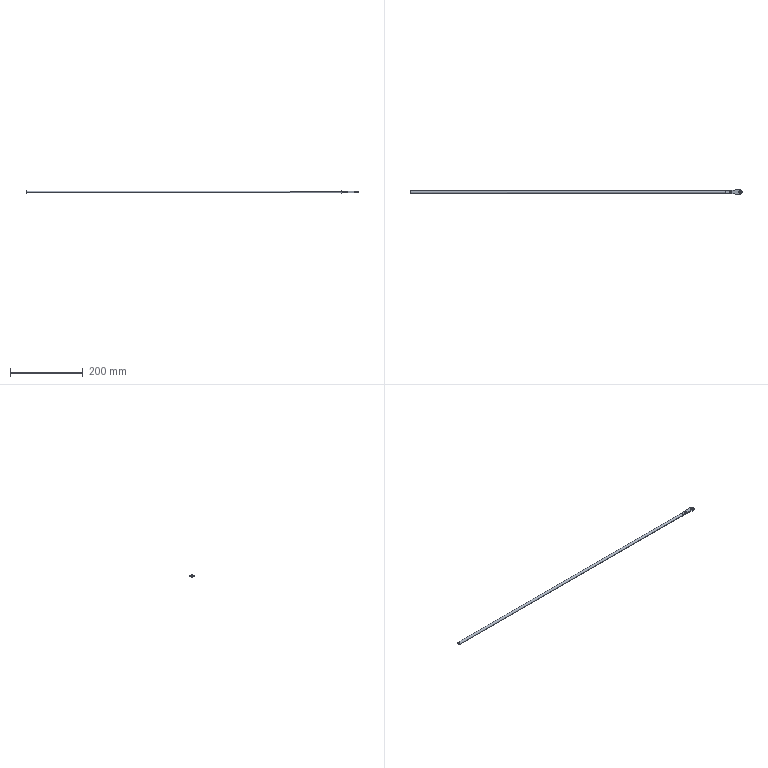Component | SolidWorks | RightRearDoorFrameAssembly-1_RearDoorUpperLockRod-1 | 1 solid | 20 faces | box 912.5 x 13 x 8 mm | volume 44809 mm3 | plane 11 | cylinder 7 | cone 2 | commonest cylinder face diameters 6.5 x4 8 x2 13 x1
build123d program:
from build123d import *

# Parameters (mm, degrees)
SKETCH1_R           = 4
BOSS_EXTRUDE1_DEPTH = 912.5
CUT_EXTRUDE1_DEPTH  = 5
SKETCH3_W           = 42
SKETCH3_H           = 2.024
CUT_EXTRUDE2_DEPTH  = 10
BOSS_EXTRUDE2_DEPTH = 3
CUT_EXTRUDE3_DEPTH  = 3
SKETCH6_R           = 3.25
CUT_EXTRUDE4_DEPTH  = 3
CHAMFER1_SIZE       = 1.5


with BuildPart() as part:
    # Sketch1 → Boss-Extrude1 (new body)
    with BuildSketch(Plane(origin=(0, 0, 0), x_dir=(0, 0, -1), z_dir=(1, 0, 0))):
        Circle(SKETCH1_R)
    extrude(amount=-BOSS_EXTRUDE1_DEPTH)

    # Sketch2 → Cut-Extrude1 (cut, symmetric)
    with BuildSketch(Plane.XY):
        Polygon((-42, 1.5), (-45.678, 4), (-42, 4), (0, 4), (0, 1.5), align=None)
        Polygon((-45.678, -4), (-42, -4), (0, -4), (0, -1.5), (-42, -1.5), align=None)
    extrude(amount=CUT_EXTRUDE1_DEPTH, both=True, mode=Mode.SUBTRACT)

    # Sketch3 → Cut-Extrude2 (cut)
    with BuildSketch(Plane(origin=(0, 1.5, 0), x_dir=(1, 0, 0), z_dir=(0, 1, 0))):
        with Locations((-21, 2.988)):
            Rectangle(SKETCH3_W, SKETCH3_H)
        with Locations((-21, -2.988)):
            Rectangle(SKETCH3_W, SKETCH3_H)
    extrude(amount=-CUT_EXTRUDE2_DEPTH, mode=Mode.SUBTRACT)

    # Sketch4 → Boss-Extrude2 (add)
    with BuildSketch(Plane(origin=(0, 1.5, 0), x_dir=(1, 0, 0), z_dir=(0, 1, 0))):
        with BuildLine():
            Line((-42, -4), (-42, 4))
            Line((-42, 4), (-7.386, 6.439))
            ThreePointArc((-7.386, 6.439), (0, 0), (-7.386, -6.439))
            Line((-7.386, -6.439), (-42, -4))
        make_face()
    extrude(amount=-BOSS_EXTRUDE2_DEPTH)

    # Sketch5 → Cut-Extrude3 (cut)
    with BuildSketch(Plane(origin=(0, 1.5, 0), x_dir=(1, 0, 0), z_dir=(0, 1, 0))):
        with BuildLine():
            Line((-0.8017, 3.127), (2.344, 3.127))
            Line((2.344, 3.127), (2.344, -3.404))
            Line((2.344, -3.404), (-0.9628, -3.404))
            ThreePointArc((-0.9628, -3.404), (-0.001977, -0.1603), (-0.8017, 3.127))
        make_face()
    extrude(amount=-CUT_EXTRUDE3_DEPTH, mode=Mode.SUBTRACT)

    # Sketch6 → Cut-Extrude4 (cut)
    with BuildSketch(Plane(origin=(0, 1.5, 0), x_dir=(1, 0, 0), z_dir=(0, 1, 0))):
        with Locations(Location((-6, 0, 0), (0, 0, 180))):
            Circle(SKETCH6_R)
        with Locations(Location((-31, 0, 0), (0, 0, 180))):
            Circle(SKETCH6_R)
    extrude(amount=-CUT_EXTRUDE4_DEPTH, mode=Mode.SUBTRACT)

    # Chamfer1
    chamfer1_edges = [part.edges().sort_by_distance(p)[0] for p in [
        (-912.5, 0, 4),
    ]]
    chamfer(chamfer1_edges, length=CHAMFER1_SIZE)


solid = part.part

# Placed as in the assembly
solid = solid.moved(Location((-209.186, 303.707, -28.746), (90, 0, 0)))
STEP:
#1=COLOUR_RGB('',0.7922,0.8196,0.9333);
#2=FILL_AREA_STYLE_COLOUR('',#1);
#3=FILL_AREA_STYLE('',(#2));
#4=SURFACE_STYLE_FILL_AREA(#3);
#5=SURFACE_SIDE_STYLE('',(#4));
#6=SURFACE_STYLE_USAGE(.BOTH.,#5);
#7=PRESENTATION_STYLE_ASSIGNMENT((#6));
#8=CARTESIAN_POINT('',(-44.161,12.055,-1.132));
#9=VERTEX_POINT('',#8);
#10=CARTESIAN_POINT('',(-44.161,11.859,-1.132));
#11=VERTEX_POINT('',#10);
#12=CARTESIAN_POINT('',(-44.161,11.957,-1.132));
#13=DIRECTION('',(-1.,-0.,-0.));
#14=DIRECTION('',(0.,-1.,0.));
#15=AXIS2_PLACEMENT_3D('',#12,#13,#14);
#16=CIRCLE('',#15,0.09843);
#17=EDGE_CURVE('',#9,#11,#16,.T.);
#18=ORIENTED_EDGE('',*,*,#17,.F.);
#19=CARTESIAN_POINT('',(-44.102,12.114,-1.132));
#20=VERTEX_POINT('',#19);
#21=CARTESIAN_POINT('',(-44.102,12.114,-1.132));
#22=DIRECTION('',(0.7071,0.7071,0.));
#23=VECTOR('',#22,39.37);
#24=LINE('',#21,#23);
#25=EDGE_CURVE('',#9,#20,#24,.T.);
#26=ORIENTED_EDGE('',*,*,#25,.T.);
#27=CARTESIAN_POINT('',(-44.102,11.799,-1.132));
#28=VERTEX_POINT('',#27);
#29=CARTESIAN_POINT('',(-44.102,11.957,-1.132));
#30=DIRECTION('',(1.,0.,0.));
#31=DIRECTION('',(0.,-1.,0.));
#32=AXIS2_PLACEMENT_3D('',#29,#30,#31);
#33=CIRCLE('',#32,0.1575);
#34=EDGE_CURVE('',#28,#20,#33,.T.);
#35=ORIENTED_EDGE('',*,*,#34,.F.);
#36=CARTESIAN_POINT('',(-44.102,11.799,-1.132));
#37=DIRECTION('',(0.7071,-0.7071,0.));
#38=VECTOR('',#37,39.37);
#39=LINE('',#36,#38);
#40=EDGE_CURVE('',#11,#28,#39,.T.);
#41=ORIENTED_EDGE('',*,*,#40,.F.);
#42=EDGE_LOOP('',(#18,#26,#35,#41));
#43=FACE_OUTER_BOUND('',#42,.T.);
#44=CARTESIAN_POINT('',(-44.102,11.957,-1.132));
#45=DIRECTION('',(1.,0.,0.));
#46=DIRECTION('',(0.,-1.,0.));
#47=AXIS2_PLACEMENT_3D('',#44,#45,#46);
#48=CONICAL_SURFACE('',#47,0.1575,0.7854);
#49=ADVANCED_FACE('',(#43),#48,.T.);
#50=CARTESIAN_POINT('',(-9.328,11.957,-1.073));
#51=VERTEX_POINT('',#50);
#52=CARTESIAN_POINT('',(-9.584,11.957,-1.073));
#53=VERTEX_POINT('',#52);
#54=CARTESIAN_POINT('',(-9.456,11.957,-1.073));
#55=DIRECTION('',(0.,0.,-1.));
#56=DIRECTION('',(-1.,0.,0.));
#57=AXIS2_PLACEMENT_3D('',#54,#55,#56);
#58=CIRCLE('',#57,0.128);
#59=EDGE_CURVE('',#51,#53,#58,.T.);
#60=ORIENTED_EDGE('',*,*,#59,.F.);
#61=CARTESIAN_POINT('',(-9.328,11.957,-1.191));
#62=VERTEX_POINT('',#61);
#63=CARTESIAN_POINT('',(-9.328,11.957,-1.073));
#64=DIRECTION('',(0.,0.,-1.));
#65=VECTOR('',#64,39.37);
#66=LINE('',#63,#65);
#67=EDGE_CURVE('',#51,#62,#66,.T.);
#68=ORIENTED_EDGE('',*,*,#67,.T.);
#69=CARTESIAN_POINT('',(-9.584,11.957,-1.191));
#70=VERTEX_POINT('',#69);
#71=CARTESIAN_POINT('',(-9.456,11.957,-1.191));
#72=DIRECTION('',(0.,0.,-1.));
#73=DIRECTION('',(-1.,0.,0.));
#74=AXIS2_PLACEMENT_3D('',#71,#72,#73);
#75=CIRCLE('',#74,0.128);
#76=EDGE_CURVE('',#62,#70,#75,.T.);
#77=ORIENTED_EDGE('',*,*,#76,.T.);
#78=CARTESIAN_POINT('',(-9.584,11.957,-1.073));
#79=DIRECTION('',(0.,0.,-1.));
#80=VECTOR('',#79,39.37);
#81=LINE('',#78,#80);
#82=EDGE_CURVE('',#53,#70,#81,.T.);
#83=ORIENTED_EDGE('',*,*,#82,.F.);
#84=EDGE_LOOP('',(#60,#68,#77,#83));
#85=FACE_OUTER_BOUND('',#84,.T.);
#86=CARTESIAN_POINT('',(-9.456,11.957,-1.073));
#87=DIRECTION('',(0.,0.,-1.));
#88=DIRECTION('',(-1.,0.,0.));
#89=AXIS2_PLACEMENT_3D('',#86,#87,#88);
#90=CYLINDRICAL_SURFACE('',#89,0.128);
#91=ADVANCED_FACE('',(#85),#90,.F.);
#92=CARTESIAN_POINT('',(-8.344,11.957,-1.073));
#93=VERTEX_POINT('',#92);
#94=CARTESIAN_POINT('',(-8.6,11.957,-1.073));
#95=VERTEX_POINT('',#94);
#96=CARTESIAN_POINT('',(-8.472,11.957,-1.073));
#97=DIRECTION('',(0.,0.,-1.));
#98=DIRECTION('',(-1.,0.,0.));
#99=AXIS2_PLACEMENT_3D('',#96,#97,#98);
#100=CIRCLE('',#99,0.128);
#101=EDGE_CURVE('',#93,#95,#100,.T.);
#102=ORIENTED_EDGE('',*,*,#101,.F.);
#103=CARTESIAN_POINT('',(-8.344,11.957,-1.191));
#104=VERTEX_POINT('',#103);
#105=CARTESIAN_POINT('',(-8.344,11.957,-1.073));
#106=DIRECTION('',(0.,0.,-1.));
#107=VECTOR('',#106,39.37);
#108=LINE('',#105,#107);
#109=EDGE_CURVE('',#93,#104,#108,.T.);
#110=ORIENTED_EDGE('',*,*,#109,.T.);
#111=CARTESIAN_POINT('',(-8.6,11.957,-1.191));
#112=VERTEX_POINT('',#111);
#113=CARTESIAN_POINT('',(-8.472,11.957,-1.191));
#114=DIRECTION('',(0.,0.,-1.));
#115=DIRECTION('',(-1.,0.,0.));
#116=AXIS2_PLACEMENT_3D('',#113,#114,#115);
#117=CIRCLE('',#116,0.128);
#118=EDGE_CURVE('',#104,#112,#117,.T.);
#119=ORIENTED_EDGE('',*,*,#118,.T.);
#120=CARTESIAN_POINT('',(-8.6,11.957,-1.073));
#121=DIRECTION('',(0.,0.,-1.));
#122=VECTOR('',#121,39.37);
#123=LINE('',#120,#122);
#124=EDGE_CURVE('',#95,#112,#123,.T.);
#125=ORIENTED_EDGE('',*,*,#124,.F.);
#126=EDGE_LOOP('',(#102,#110,#119,#125));
#127=FACE_OUTER_BOUND('',#126,.T.);
#128=CARTESIAN_POINT('',(-8.472,11.957,-1.073));
#129=DIRECTION('',(0.,0.,-1.));
#130=DIRECTION('',(-1.,0.,0.));
#131=AXIS2_PLACEMENT_3D('',#128,#129,#130);
#132=CYLINDRICAL_SURFACE('',#131,0.128);
#133=ADVANCED_FACE('',(#127),#132,.F.);
#134=ORIENTED_EDGE('',*,*,#34,.T.);
#135=CARTESIAN_POINT('',(-9.889,12.114,-1.132));
#136=VERTEX_POINT('',#135);
#137=CARTESIAN_POINT('',(-44.161,12.114,-1.132));
#138=DIRECTION('',(1.,0.,0.));
#139=VECTOR('',#138,39.37);
#140=LINE('',#137,#139);
#141=EDGE_CURVE('',#20,#136,#140,.T.);
#142=ORIENTED_EDGE('',*,*,#141,.T.);
#143=CARTESIAN_POINT('',(-9.889,12.103,-1.191));
#144=VERTEX_POINT('',#143);
#145=CARTESIAN_POINT('',(-9.889,11.957,-1.132));
#146=DIRECTION('',(1.,0.,0.));
#147=DIRECTION('',(0.,-0.,1.));
#148=AXIS2_PLACEMENT_3D('',#145,#146,#147);
#149=CIRCLE('',#148,0.1575);
#150=EDGE_CURVE('',#144,#136,#149,.T.);
#151=ORIENTED_EDGE('',*,*,#150,.F.);
#152=CARTESIAN_POINT('',(-9.889,11.811,-1.191));
#153=VERTEX_POINT('',#152);
#154=CARTESIAN_POINT('',(-9.889,11.811,-1.191));
#155=CARTESIAN_POINT('',(-10.117,11.874,-1.345));
#156=CARTESIAN_POINT('',(-10.117,12.04,-1.345));
#157=CARTESIAN_POINT('',(-9.889,12.103,-1.191));
#158=(BOUNDED_CURVE()B_SPLINE_CURVE(3,(#154,#155,#156,#157),.UNSPECIFIED.,.F.,.T.)B_SPLINE_CURVE_WITH_KNOTS((4,4),(1.955,4.328),.UNSPECIFIED.)CURVE()GEOMETRIC_REPRESENTATION_ITEM()RATIONAL_B_SPLINE_CURVE((1.,0.5833,0.5833,1.))REPRESENTATION_ITEM(''));
#159=EDGE_CURVE('',#153,#144,#158,.T.);
#160=ORIENTED_EDGE('',*,*,#159,.F.);
#161=CARTESIAN_POINT('',(-9.889,11.799,-1.132));
#162=VERTEX_POINT('',#161);
#163=CARTESIAN_POINT('',(-9.889,11.957,-1.132));
#164=DIRECTION('',(1.,0.,0.));
#165=DIRECTION('',(0.,-0.,1.));
#166=AXIS2_PLACEMENT_3D('',#163,#164,#165);
#167=CIRCLE('',#166,0.1575);
#168=EDGE_CURVE('',#162,#153,#167,.T.);
#169=ORIENTED_EDGE('',*,*,#168,.F.);
#170=CARTESIAN_POINT('',(-44.161,11.799,-1.132));
#171=DIRECTION('',(1.,0.,0.));
#172=VECTOR('',#171,39.37);
#173=LINE('',#170,#172);
#174=EDGE_CURVE('',#28,#162,#173,.T.);
#175=ORIENTED_EDGE('',*,*,#174,.F.);
#176=EDGE_LOOP('',(#134,#142,#151,#160,#169,#175));
#177=FACE_OUTER_BOUND('',#176,.T.);
#178=CARTESIAN_POINT('',(-44.161,11.957,-1.132));
#179=DIRECTION('',(1.,0.,0.));
#180=DIRECTION('',(0.,-1.,0.));
#181=AXIS2_PLACEMENT_3D('',#178,#179,#180);
#182=CYLINDRICAL_SURFACE('',#181,0.1575);
#183=ADVANCED_FACE('',(#177),#182,.T.);
#184=ORIENTED_EDGE('',*,*,#141,.F.);
#185=CARTESIAN_POINT('',(-44.102,11.957,-1.132));
#186=DIRECTION('',(1.,0.,0.));
#187=DIRECTION('',(0.,-1.,0.));
#188=AXIS2_PLACEMENT_3D('',#185,#186,#187);
#189=CIRCLE('',#188,0.1575);
#190=EDGE_CURVE('',#20,#28,#189,.T.);
#191=ORIENTED_EDGE('',*,*,#190,.T.);
#192=ORIENTED_EDGE('',*,*,#174,.T.);
#193=CARTESIAN_POINT('',(-9.889,11.811,-1.073));
#194=VERTEX_POINT('',#193);
#195=CARTESIAN_POINT('',(-9.889,11.957,-1.132));
#196=DIRECTION('',(1.,0.,0.));
#197=DIRECTION('',(0.,-0.,1.));
#198=AXIS2_PLACEMENT_3D('',#195,#196,#197);
#199=CIRCLE('',#198,0.1575);
#200=EDGE_CURVE('',#194,#162,#199,.T.);
#201=ORIENTED_EDGE('',*,*,#200,.F.);
#202=CARTESIAN_POINT('',(-9.889,12.103,-1.073));
#203=VERTEX_POINT('',#202);
#204=CARTESIAN_POINT('',(-9.889,12.103,-1.073));
#205=CARTESIAN_POINT('',(-10.117,12.04,-0.918));
#206=CARTESIAN_POINT('',(-10.117,11.874,-0.918));
#207=CARTESIAN_POINT('',(-9.889,11.811,-1.073));
#208=(BOUNDED_CURVE()B_SPLINE_CURVE(3,(#204,#205,#206,#207),.UNSPECIFIED.,.F.,.F.)B_SPLINE_CURVE_WITH_KNOTS((4,4),(1.955,4.328),.UNSPECIFIED.)CURVE()GEOMETRIC_REPRESENTATION_ITEM()RATIONAL_B_SPLINE_CURVE((1.,0.5833,0.5833,1.))REPRESENTATION_ITEM(''));
#209=EDGE_CURVE('',#203,#194,#208,.T.);
#210=ORIENTED_EDGE('',*,*,#209,.F.);
#211=CARTESIAN_POINT('',(-9.889,11.957,-1.132));
#212=DIRECTION('',(1.,0.,0.));
#213=DIRECTION('',(0.,0.,1.));
#214=AXIS2_PLACEMENT_3D('',#211,#212,#213);
#215=CIRCLE('',#214,0.1575);
#216=EDGE_CURVE('',#136,#203,#215,.T.);
#217=ORIENTED_EDGE('',*,*,#216,.F.);
#218=EDGE_LOOP('',(#184,#191,#192,#201,#210,#217));
#219=FACE_OUTER_BOUND('',#218,.T.);
#220=CARTESIAN_POINT('',(-44.161,11.957,-1.132));
#221=DIRECTION('',(1.,0.,0.));
#222=DIRECTION('',(0.,-1.,0.));
#223=AXIS2_PLACEMENT_3D('',#220,#221,#222);
#224=CYLINDRICAL_SURFACE('',#223,0.1575);
#225=ADVANCED_FACE('',(#219),#224,.T.);
#226=CARTESIAN_POINT('',(-44.161,11.957,-1.132));
#227=DIRECTION('',(-1.,-0.,-0.));
#228=DIRECTION('',(0.,-1.,0.));
#229=AXIS2_PLACEMENT_3D('',#226,#227,#228);
#230=CIRCLE('',#229,0.09843);
#231=EDGE_CURVE('',#11,#9,#230,.T.);
#232=ORIENTED_EDGE('',*,*,#231,.T.);
#233=ORIENTED_EDGE('',*,*,#17,.T.);
#234=EDGE_LOOP('',(#232,#233));
#235=FACE_OUTER_BOUND('',#234,.T.);
#236=CARTESIAN_POINT('',(-44.161,11.957,-1.132));
#237=DIRECTION('',(1.,0.,0.));
#238=DIRECTION('',(0.,-1.,-0.));
#239=AXIS2_PLACEMENT_3D('',#236,#237,#238);
#240=PLANE('',#239);
#241=ADVANCED_FACE('',(#235),#240,.F.);
#242=CARTESIAN_POINT('',(-9.456,11.957,-1.191));
#243=DIRECTION('',(0.,0.,-1.));
#244=DIRECTION('',(-1.,0.,0.));
#245=AXIS2_PLACEMENT_3D('',#242,#243,#244);
#246=CIRCLE('',#245,0.128);
#247=EDGE_CURVE('',#70,#62,#246,.T.);
#248=ORIENTED_EDGE('',*,*,#247,.F.);
#249=ORIENTED_EDGE('',*,*,#76,.F.);
#250=EDGE_LOOP('',(#248,#249));
#251=FACE_BOUND('',#250,.T.);
#252=CARTESIAN_POINT('',(-8.472,11.957,-1.191));
#253=DIRECTION('',(0.,0.,-1.));
#254=DIRECTION('',(-1.,0.,0.));
#255=AXIS2_PLACEMENT_3D('',#252,#253,#254);
#256=CIRCLE('',#255,0.128);
#257=EDGE_CURVE('',#112,#104,#256,.T.);
#258=ORIENTED_EDGE('',*,*,#257,.F.);
#259=ORIENTED_EDGE('',*,*,#118,.F.);
#260=EDGE_LOOP('',(#258,#259));
#261=FACE_BOUND('',#260,.T.);
#262=CARTESIAN_POINT('',(-9.889,12.114,-1.191));
#263=VERTEX_POINT('',#262);
#264=CARTESIAN_POINT('',(-8.526,12.21,-1.191));
#265=VERTEX_POINT('',#264);
#266=CARTESIAN_POINT('',(-9.889,12.114,-1.191));
#267=DIRECTION('',(0.9975,0.0703,0.));
#268=VECTOR('',#267,39.37);
#269=LINE('',#266,#268);
#270=EDGE_CURVE('',#263,#265,#269,.T.);
#271=ORIENTED_EDGE('',*,*,#270,.T.);
#272=CARTESIAN_POINT('',(-8.526,11.703,-1.191));
#273=VERTEX_POINT('',#272);
#274=CARTESIAN_POINT('',(-8.492,11.957,-1.191));
#275=DIRECTION('',(0.,0.,-1.));
#276=DIRECTION('',(-1.,0.,0.));
#277=AXIS2_PLACEMENT_3D('',#274,#275,#276);
#278=CIRCLE('',#277,0.2559);
#279=EDGE_CURVE('',#265,#273,#278,.T.);
#280=ORIENTED_EDGE('',*,*,#279,.T.);
#281=CARTESIAN_POINT('',(-9.889,11.799,-1.191));
#282=VERTEX_POINT('',#281);
#283=CARTESIAN_POINT('',(-9.889,11.799,-1.191));
#284=DIRECTION('',(-0.9975,0.0703,-0.));
#285=VECTOR('',#284,39.37);
#286=LINE('',#283,#285);
#287=EDGE_CURVE('',#273,#282,#286,.T.);
#288=ORIENTED_EDGE('',*,*,#287,.T.);
#289=CARTESIAN_POINT('',(-9.889,12.114,-1.191));
#290=DIRECTION('',(-0.,1.,0.));
#291=VECTOR('',#290,39.37);
#292=LINE('',#289,#291);
#293=EDGE_CURVE('',#282,#153,#292,.T.);
#294=ORIENTED_EDGE('',*,*,#293,.T.);
#295=CARTESIAN_POINT('',(-9.889,11.76,-1.191));
#296=DIRECTION('',(-0.,1.,0.));
#297=VECTOR('',#296,39.37);
#298=LINE('',#295,#297);
#299=EDGE_CURVE('',#153,#144,#298,.T.);
#300=ORIENTED_EDGE('',*,*,#299,.T.);
#301=CARTESIAN_POINT('',(-9.889,12.114,-1.191));
#302=DIRECTION('',(-0.,1.,0.));
#303=VECTOR('',#302,39.37);
#304=LINE('',#301,#303);
#305=EDGE_CURVE('',#144,#263,#304,.T.);
#306=ORIENTED_EDGE('',*,*,#305,.T.);
#307=EDGE_LOOP('',(#271,#280,#288,#294,#300,#306));
#308=FACE_OUTER_BOUND('',#307,.T.);
#309=CARTESIAN_POINT('',(-8.236,11.76,-1.191));
#310=DIRECTION('',(-0.,-0.,1.));
#311=DIRECTION('',(1.,0.,0.));
#312=AXIS2_PLACEMENT_3D('',#309,#310,#311);
#313=PLANE('',#312);
#314=ADVANCED_FACE('',(#251,#261,#308),#313,.F.);
#315=ORIENTED_EDGE('',*,*,#299,.F.);
#316=ORIENTED_EDGE('',*,*,#159,.T.);
#317=EDGE_LOOP('',(#315,#316));
#318=FACE_OUTER_BOUND('',#317,.T.);
#319=CARTESIAN_POINT('',(-9.889,11.76,-1.191));
#320=DIRECTION('',(-0.5621,-0.,0.8271));
#321=DIRECTION('',(0.8271,0.,0.5621));
#322=AXIS2_PLACEMENT_3D('',#319,#320,#321);
#323=PLANE('',#322);
#324=ADVANCED_FACE('',(#318),#323,.F.);
#325=CARTESIAN_POINT('',(-9.889,11.76,-1.073));
#326=DIRECTION('',(-0.,1.,0.));
#327=VECTOR('',#326,39.37);
#328=LINE('',#325,#327);
#329=EDGE_CURVE('',#194,#203,#328,.T.);
#330=ORIENTED_EDGE('',*,*,#329,.T.);
#331=ORIENTED_EDGE('',*,*,#209,.T.);
#332=EDGE_LOOP('',(#330,#331));
#333=FACE_OUTER_BOUND('',#332,.T.);
#334=CARTESIAN_POINT('',(-9.889,11.76,-1.073));
#335=DIRECTION('',(-0.5621,-0.,-0.8271));
#336=DIRECTION('',(-0.8271,-0.,0.5621));
#337=AXIS2_PLACEMENT_3D('',#334,#335,#336);
#338=PLANE('',#337);
#339=ADVANCED_FACE('',(#333),#338,.F.);
#340=CARTESIAN_POINT('',(-9.456,11.957,-1.073));
#341=DIRECTION('',(0.,0.,-1.));
#342=DIRECTION('',(-1.,0.,0.));
#343=AXIS2_PLACEMENT_3D('',#340,#341,#342);
#344=CIRCLE('',#343,0.128);
#345=EDGE_CURVE('',#53,#51,#344,.T.);
#346=ORIENTED_EDGE('',*,*,#345,.T.);
#347=ORIENTED_EDGE('',*,*,#59,.T.);
#348=EDGE_LOOP('',(#346,#347));
#349=FACE_BOUND('',#348,.T.);
#350=CARTESIAN_POINT('',(-8.472,11.957,-1.073));
#351=DIRECTION('',(0.,0.,-1.));
#352=DIRECTION('',(-1.,0.,0.));
#353=AXIS2_PLACEMENT_3D('',#350,#351,#352);
#354=CIRCLE('',#353,0.128);
#355=EDGE_CURVE('',#95,#93,#354,.T.);
#356=ORIENTED_EDGE('',*,*,#355,.T.);
#357=ORIENTED_EDGE('',*,*,#101,.T.);
#358=EDGE_LOOP('',(#356,#357));
#359=FACE_BOUND('',#358,.T.);
#360=CARTESIAN_POINT('',(-8.526,12.21,-1.073));
#361=VERTEX_POINT('',#360);
#362=CARTESIAN_POINT('',(-8.526,11.703,-1.073));
#363=VERTEX_POINT('',#362);
#364=CARTESIAN_POINT('',(-8.492,11.957,-1.073));
#365=DIRECTION('',(0.,0.,-1.));
#366=DIRECTION('',(-1.,0.,0.));
#367=AXIS2_PLACEMENT_3D('',#364,#365,#366);
#368=CIRCLE('',#367,0.2559);
#369=EDGE_CURVE('',#361,#363,#368,.T.);
#370=ORIENTED_EDGE('',*,*,#369,.F.);
#371=CARTESIAN_POINT('',(-9.889,12.114,-1.073));
#372=VERTEX_POINT('',#371);
#373=CARTESIAN_POINT('',(-9.889,12.114,-1.073));
#374=DIRECTION('',(0.9975,0.0703,0.));
#375=VECTOR('',#374,39.37);
#376=LINE('',#373,#375);
#377=EDGE_CURVE('',#372,#361,#376,.T.);
#378=ORIENTED_EDGE('',*,*,#377,.F.);
#379=CARTESIAN_POINT('',(-9.889,12.114,-1.073));
#380=DIRECTION('',(-0.,1.,0.));
#381=VECTOR('',#380,39.37);
#382=LINE('',#379,#381);
#383=EDGE_CURVE('',#203,#372,#382,.T.);
#384=ORIENTED_EDGE('',*,*,#383,.F.);
#385=ORIENTED_EDGE('',*,*,#329,.F.);
#386=CARTESIAN_POINT('',(-9.889,11.799,-1.073));
#387=VERTEX_POINT('',#386);
#388=CARTESIAN_POINT('',(-9.889,12.114,-1.073));
#389=DIRECTION('',(-0.,1.,0.));
#390=VECTOR('',#389,39.37);
#391=LINE('',#388,#390);
#392=EDGE_CURVE('',#387,#194,#391,.T.);
#393=ORIENTED_EDGE('',*,*,#392,.F.);
#394=CARTESIAN_POINT('',(-9.889,11.799,-1.073));
#395=DIRECTION('',(-0.9975,0.0703,-0.));
#396=VECTOR('',#395,39.37);
#397=LINE('',#394,#396);
#398=EDGE_CURVE('',#363,#387,#397,.T.);
#399=ORIENTED_EDGE('',*,*,#398,.F.);
#400=EDGE_LOOP('',(#370,#378,#384,#385,#393,#399));
#401=FACE_OUTER_BOUND('',#400,.T.);
#402=CARTESIAN_POINT('',(-8.236,11.76,-1.073));
#403=DIRECTION('',(0.,0.,-1.));
#404=DIRECTION('',(-1.,-0.,-0.));
#405=AXIS2_PLACEMENT_3D('',#402,#403,#404);
#406=PLANE('',#405);
#407=ADVANCED_FACE('',(#349,#359,#401),#406,.F.);
#408=ORIENTED_EDGE('',*,*,#270,.F.);
#409=CARTESIAN_POINT('',(-9.889,12.114,-1.073));
#410=DIRECTION('',(0.,0.,-1.));
#411=VECTOR('',#410,39.37);
#412=LINE('',#409,#411);
#413=EDGE_CURVE('',#136,#263,#412,.T.);
#414=ORIENTED_EDGE('',*,*,#413,.F.);
#415=CARTESIAN_POINT('',(-9.889,12.114,-1.073));
#416=DIRECTION('',(0.,0.,-1.));
#417=VECTOR('',#416,39.37);
#418=LINE('',#415,#417);
#419=EDGE_CURVE('',#372,#136,#418,.T.);
#420=ORIENTED_EDGE('',*,*,#419,.F.);
#421=ORIENTED_EDGE('',*,*,#377,.T.);
#422=CARTESIAN_POINT('',(-8.526,12.21,-1.073));
#423=DIRECTION('',(0.,0.,-1.));
#424=VECTOR('',#423,39.37);
#425=LINE('',#422,#424);
#426=EDGE_CURVE('',#361,#265,#425,.T.);
#427=ORIENTED_EDGE('',*,*,#426,.T.);
#428=EDGE_LOOP('',(#408,#414,#420,#421,#427));
#429=FACE_OUTER_BOUND('',#428,.T.);
#430=CARTESIAN_POINT('',(-9.889,12.114,-1.073));
#431=DIRECTION('',(-0.0703,0.9975,0.));
#432=DIRECTION('',(0.9975,0.0703,0.));
#433=AXIS2_PLACEMENT_3D('',#430,#431,#432);
#434=PLANE('',#433);
#435=ADVANCED_FACE('',(#429),#434,.T.);
#436=ORIENTED_EDGE('',*,*,#419,.T.);
#437=ORIENTED_EDGE('',*,*,#216,.T.);
#438=ORIENTED_EDGE('',*,*,#383,.T.);
#439=EDGE_LOOP('',(#436,#437,#438));
#440=FACE_OUTER_BOUND('',#439,.T.);
#441=CARTESIAN_POINT('',(-9.889,12.114,-1.073));
#442=DIRECTION('',(-1.,-0.,-0.));
#443=DIRECTION('',(-0.,-0.,1.));
#444=AXIS2_PLACEMENT_3D('',#441,#442,#443);
#445=PLANE('',#444);
#446=ADVANCED_FACE('',(#440),#445,.T.);
#447=ORIENTED_EDGE('',*,*,#305,.F.);
#448=ORIENTED_EDGE('',*,*,#150,.T.);
#449=ORIENTED_EDGE('',*,*,#413,.T.);
#450=EDGE_LOOP('',(#447,#448,#449));
#451=FACE_OUTER_BOUND('',#450,.T.);
#452=CARTESIAN_POINT('',(-9.889,12.114,-1.073));
#453=DIRECTION('',(-1.,-0.,-0.));
#454=DIRECTION('',(-0.,-0.,1.));
#455=AXIS2_PLACEMENT_3D('',#452,#453,#454);
#456=PLANE('',#455);
#457=ADVANCED_FACE('',(#451),#456,.T.);
#458=ORIENTED_EDGE('',*,*,#392,.T.);
#459=ORIENTED_EDGE('',*,*,#200,.T.);
#460=CARTESIAN_POINT('',(-9.889,11.799,-1.073));
#461=DIRECTION('',(0.,0.,-1.));
#462=VECTOR('',#461,39.37);
#463=LINE('',#460,#462);
#464=EDGE_CURVE('',#387,#162,#463,.T.);
#465=ORIENTED_EDGE('',*,*,#464,.F.);
#466=EDGE_LOOP('',(#458,#459,#465));
#467=FACE_OUTER_BOUND('',#466,.T.);
#468=CARTESIAN_POINT('',(-9.889,12.114,-1.073));
#469=DIRECTION('',(-1.,-0.,-0.));
#470=DIRECTION('',(-0.,-0.,1.));
#471=AXIS2_PLACEMENT_3D('',#468,#469,#470);
#472=PLANE('',#471);
#473=ADVANCED_FACE('',(#467),#472,.T.);
#474=CARTESIAN_POINT('',(-9.889,11.799,-1.073));
#475=DIRECTION('',(0.,0.,-1.));
#476=VECTOR('',#475,39.37);
#477=LINE('',#474,#476);
#478=EDGE_CURVE('',#162,#282,#477,.T.);
#479=ORIENTED_EDGE('',*,*,#478,.F.);
#480=ORIENTED_EDGE('',*,*,#168,.T.);
#481=ORIENTED_EDGE('',*,*,#293,.F.);
#482=EDGE_LOOP('',(#479,#480,#481));
#483=FACE_OUTER_BOUND('',#482,.T.);
#484=CARTESIAN_POINT('',(-9.889,12.114,-1.073));
#485=DIRECTION('',(-1.,-0.,-0.));
#486=DIRECTION('',(-0.,-0.,1.));
#487=AXIS2_PLACEMENT_3D('',#484,#485,#486);
#488=PLANE('',#487);
#489=ADVANCED_FACE('',(#483),#488,.T.);
#490=CARTESIAN_POINT('',(-8.526,11.703,-1.073));
#491=DIRECTION('',(0.,0.,-1.));
#492=VECTOR('',#491,39.37);
#493=LINE('',#490,#492);
#494=EDGE_CURVE('',#363,#273,#493,.T.);
#495=ORIENTED_EDGE('',*,*,#494,.T.);
#496=ORIENTED_EDGE('',*,*,#279,.F.);
#497=ORIENTED_EDGE('',*,*,#426,.F.);
#498=ORIENTED_EDGE('',*,*,#369,.T.);
#499=EDGE_LOOP('',(#495,#496,#497,#498));
#500=FACE_OUTER_BOUND('',#499,.T.);
#501=CARTESIAN_POINT('',(-8.492,11.957,-1.073));
#502=DIRECTION('',(0.,0.,-1.));
#503=DIRECTION('',(-1.,0.,0.));
#504=AXIS2_PLACEMENT_3D('',#501,#502,#503);
#505=CYLINDRICAL_SURFACE('',#504,0.2559);
#506=ADVANCED_FACE('',(#500),#505,.T.);
#507=ORIENTED_EDGE('',*,*,#287,.F.);
#508=ORIENTED_EDGE('',*,*,#494,.F.);
#509=ORIENTED_EDGE('',*,*,#398,.T.);
#510=ORIENTED_EDGE('',*,*,#464,.T.);
#511=ORIENTED_EDGE('',*,*,#478,.T.);
#512=EDGE_LOOP('',(#507,#508,#509,#510,#511));
#513=FACE_OUTER_BOUND('',#512,.T.);
#514=CARTESIAN_POINT('',(-9.889,11.799,-1.073));
#515=DIRECTION('',(-0.0703,-0.9975,-0.));
#516=DIRECTION('',(-0.9975,0.0703,-0.));
#517=AXIS2_PLACEMENT_3D('',#514,#515,#516);
#518=PLANE('',#517);
#519=ADVANCED_FACE('',(#513),#518,.T.);
#520=ORIENTED_EDGE('',*,*,#109,.F.);
#521=ORIENTED_EDGE('',*,*,#355,.F.);
#522=ORIENTED_EDGE('',*,*,#124,.T.);
#523=ORIENTED_EDGE('',*,*,#257,.T.);
#524=EDGE_LOOP('',(#520,#521,#522,#523));
#525=FACE_OUTER_BOUND('',#524,.T.);
#526=CARTESIAN_POINT('',(-8.472,11.957,-1.073));
#527=DIRECTION('',(0.,0.,-1.));
#528=DIRECTION('',(-1.,0.,0.));
#529=AXIS2_PLACEMENT_3D('',#526,#527,#528);
#530=CYLINDRICAL_SURFACE('',#529,0.128);
#531=ADVANCED_FACE('',(#525),#530,.F.);
#532=ORIENTED_EDGE('',*,*,#67,.F.);
#533=ORIENTED_EDGE('',*,*,#345,.F.);
#534=ORIENTED_EDGE('',*,*,#82,.T.);
#535=ORIENTED_EDGE('',*,*,#247,.T.);
#536=EDGE_LOOP('',(#532,#533,#534,#535));
#537=FACE_OUTER_BOUND('',#536,.T.);
#538=CARTESIAN_POINT('',(-9.456,11.957,-1.073));
#539=DIRECTION('',(0.,0.,-1.));
#540=DIRECTION('',(-1.,0.,0.));
#541=AXIS2_PLACEMENT_3D('',#538,#539,#540);
#542=CYLINDRICAL_SURFACE('',#541,0.128);
#543=ADVANCED_FACE('',(#537),#542,.F.);
#544=ORIENTED_EDGE('',*,*,#25,.F.);
#545=ORIENTED_EDGE('',*,*,#231,.F.);
#546=ORIENTED_EDGE('',*,*,#40,.T.);
#547=ORIENTED_EDGE('',*,*,#190,.F.);
#548=EDGE_LOOP('',(#544,#545,#546,#547));
#549=FACE_OUTER_BOUND('',#548,.T.);
#550=CARTESIAN_POINT('',(-44.102,11.957,-1.132));
#551=DIRECTION('',(1.,0.,0.));
#552=DIRECTION('',(0.,-1.,0.));
#553=AXIS2_PLACEMENT_3D('',#550,#551,#552);
#554=CONICAL_SURFACE('',#553,0.1575,0.7854);
#555=ADVANCED_FACE('',(#549),#554,.T.);
#556=CLOSED_SHELL('',(#49,#91,#133,#183,#225,#241,#314,#324,#339,#407,#435,#446,#457,#473,#489,#506,#519,#531,#543,#555));
#557=MANIFOLD_SOLID_BREP('',#556);
#558=STYLED_ITEM('',(#7),#557);
#559=(LENGTH_UNIT()NAMED_UNIT(*)SI_UNIT($,.METRE.));
#560=LENGTH_MEASURE_WITH_UNIT(LENGTH_MEASURE(0.0254),#559);
#561=DIMENSIONAL_EXPONENTS(1.,0.,0.,0.,0.,0.,0.);
#562=(CONVERSION_BASED_UNIT('',#560)LENGTH_UNIT()NAMED_UNIT(#561));
#563=UNCERTAINTY_MEASURE_WITH_UNIT(LENGTH_MEASURE(0.00001),#562,'','');
#564=(NAMED_UNIT(*)PLANE_ANGLE_UNIT()SI_UNIT($,.RADIAN.));
#565=(NAMED_UNIT(*)SI_UNIT($,.STERADIAN.)SOLID_ANGLE_UNIT());
#566=(GEOMETRIC_REPRESENTATION_CONTEXT(3)GLOBAL_UNCERTAINTY_ASSIGNED_CONTEXT((#563))GLOBAL_UNIT_ASSIGNED_CONTEXT((#562,#564,#565))REPRESENTATION_CONTEXT('',''));
#567=MECHANICAL_DESIGN_GEOMETRIC_PRESENTATION_REPRESENTATION('',(#558),#566);
#568=PRESENTATION_LAYER_ASSIGNMENT('','',(#558));
#569=CARTESIAN_POINT('',(0.,0.,0.));
#570=DIRECTION('',(0.,0.,1.));
#571=DIRECTION('',(1.,0.,0.));
#572=AXIS2_PLACEMENT_3D('',#569,#570,#571);
#573=(LENGTH_UNIT()NAMED_UNIT(*)SI_UNIT($,.METRE.));
#574=LENGTH_MEASURE_WITH_UNIT(LENGTH_MEASURE(0.0254),#573);
#575=DIMENSIONAL_EXPONENTS(1.,0.,0.,0.,0.,0.,0.);
#576=(CONVERSION_BASED_UNIT('',#574)LENGTH_UNIT()NAMED_UNIT(#575));
#577=UNCERTAINTY_MEASURE_WITH_UNIT(LENGTH_MEASURE(0.00001),#576,'','');
#578=(NAMED_UNIT(*)PLANE_ANGLE_UNIT()SI_UNIT($,.RADIAN.));
#579=(NAMED_UNIT(*)SI_UNIT($,.STERADIAN.)SOLID_ANGLE_UNIT());
#580=(GEOMETRIC_REPRESENTATION_CONTEXT(3)GLOBAL_UNCERTAINTY_ASSIGNED_CONTEXT((#577))GLOBAL_UNIT_ASSIGNED_CONTEXT((#576,#578,#579))REPRESENTATION_CONTEXT('',''));
#581=ADVANCED_BREP_SHAPE_REPRESENTATION('',(#557,#572),#580);